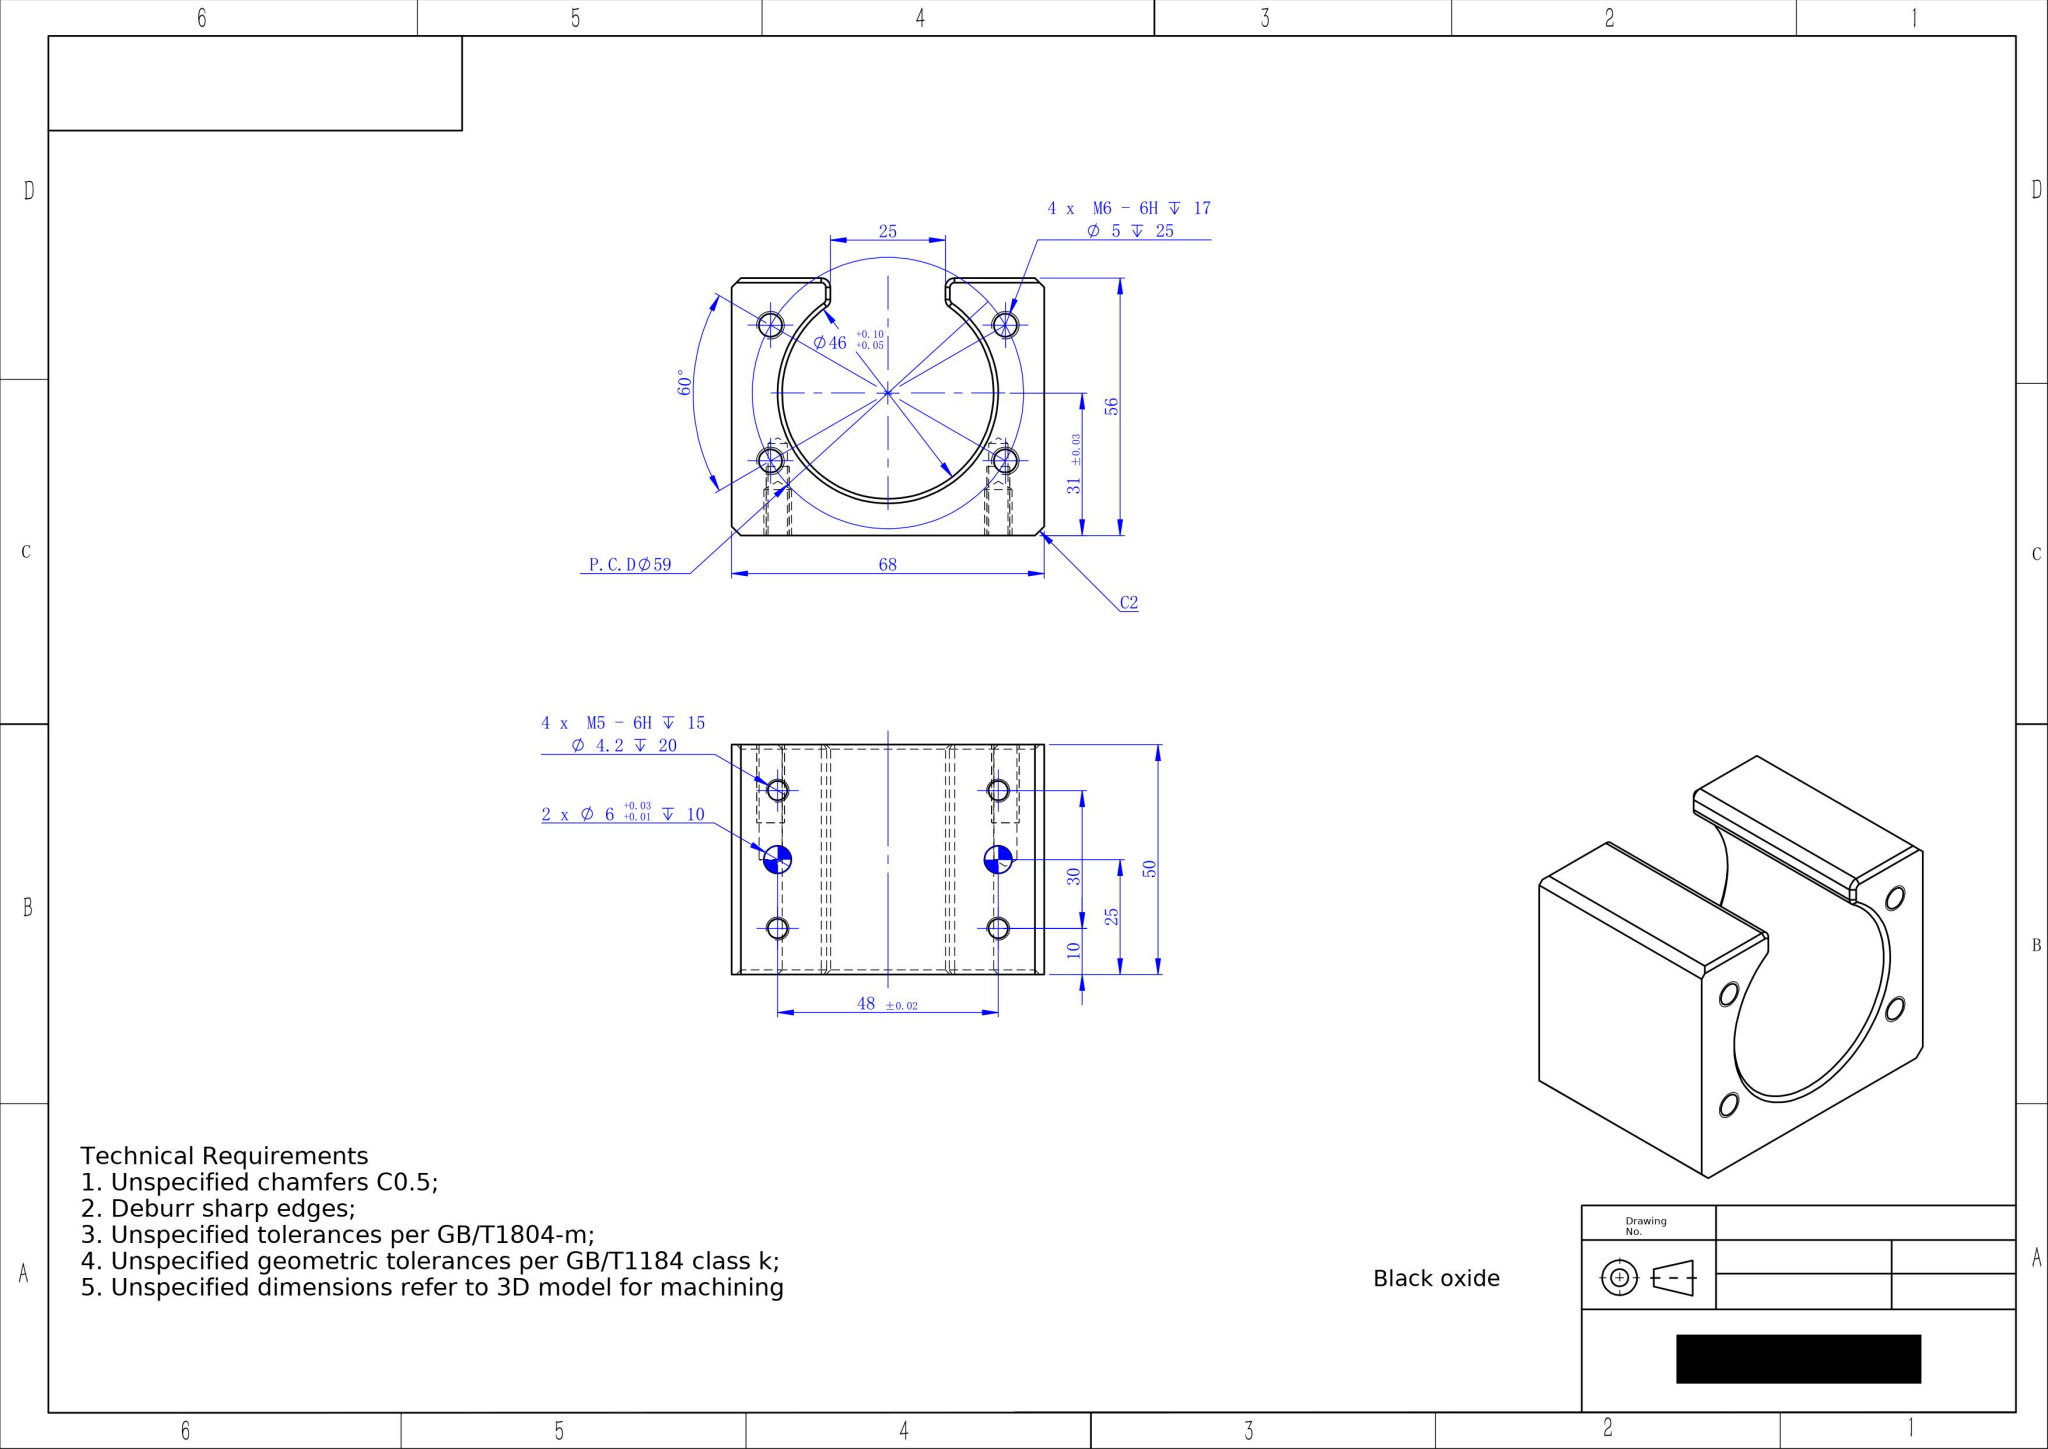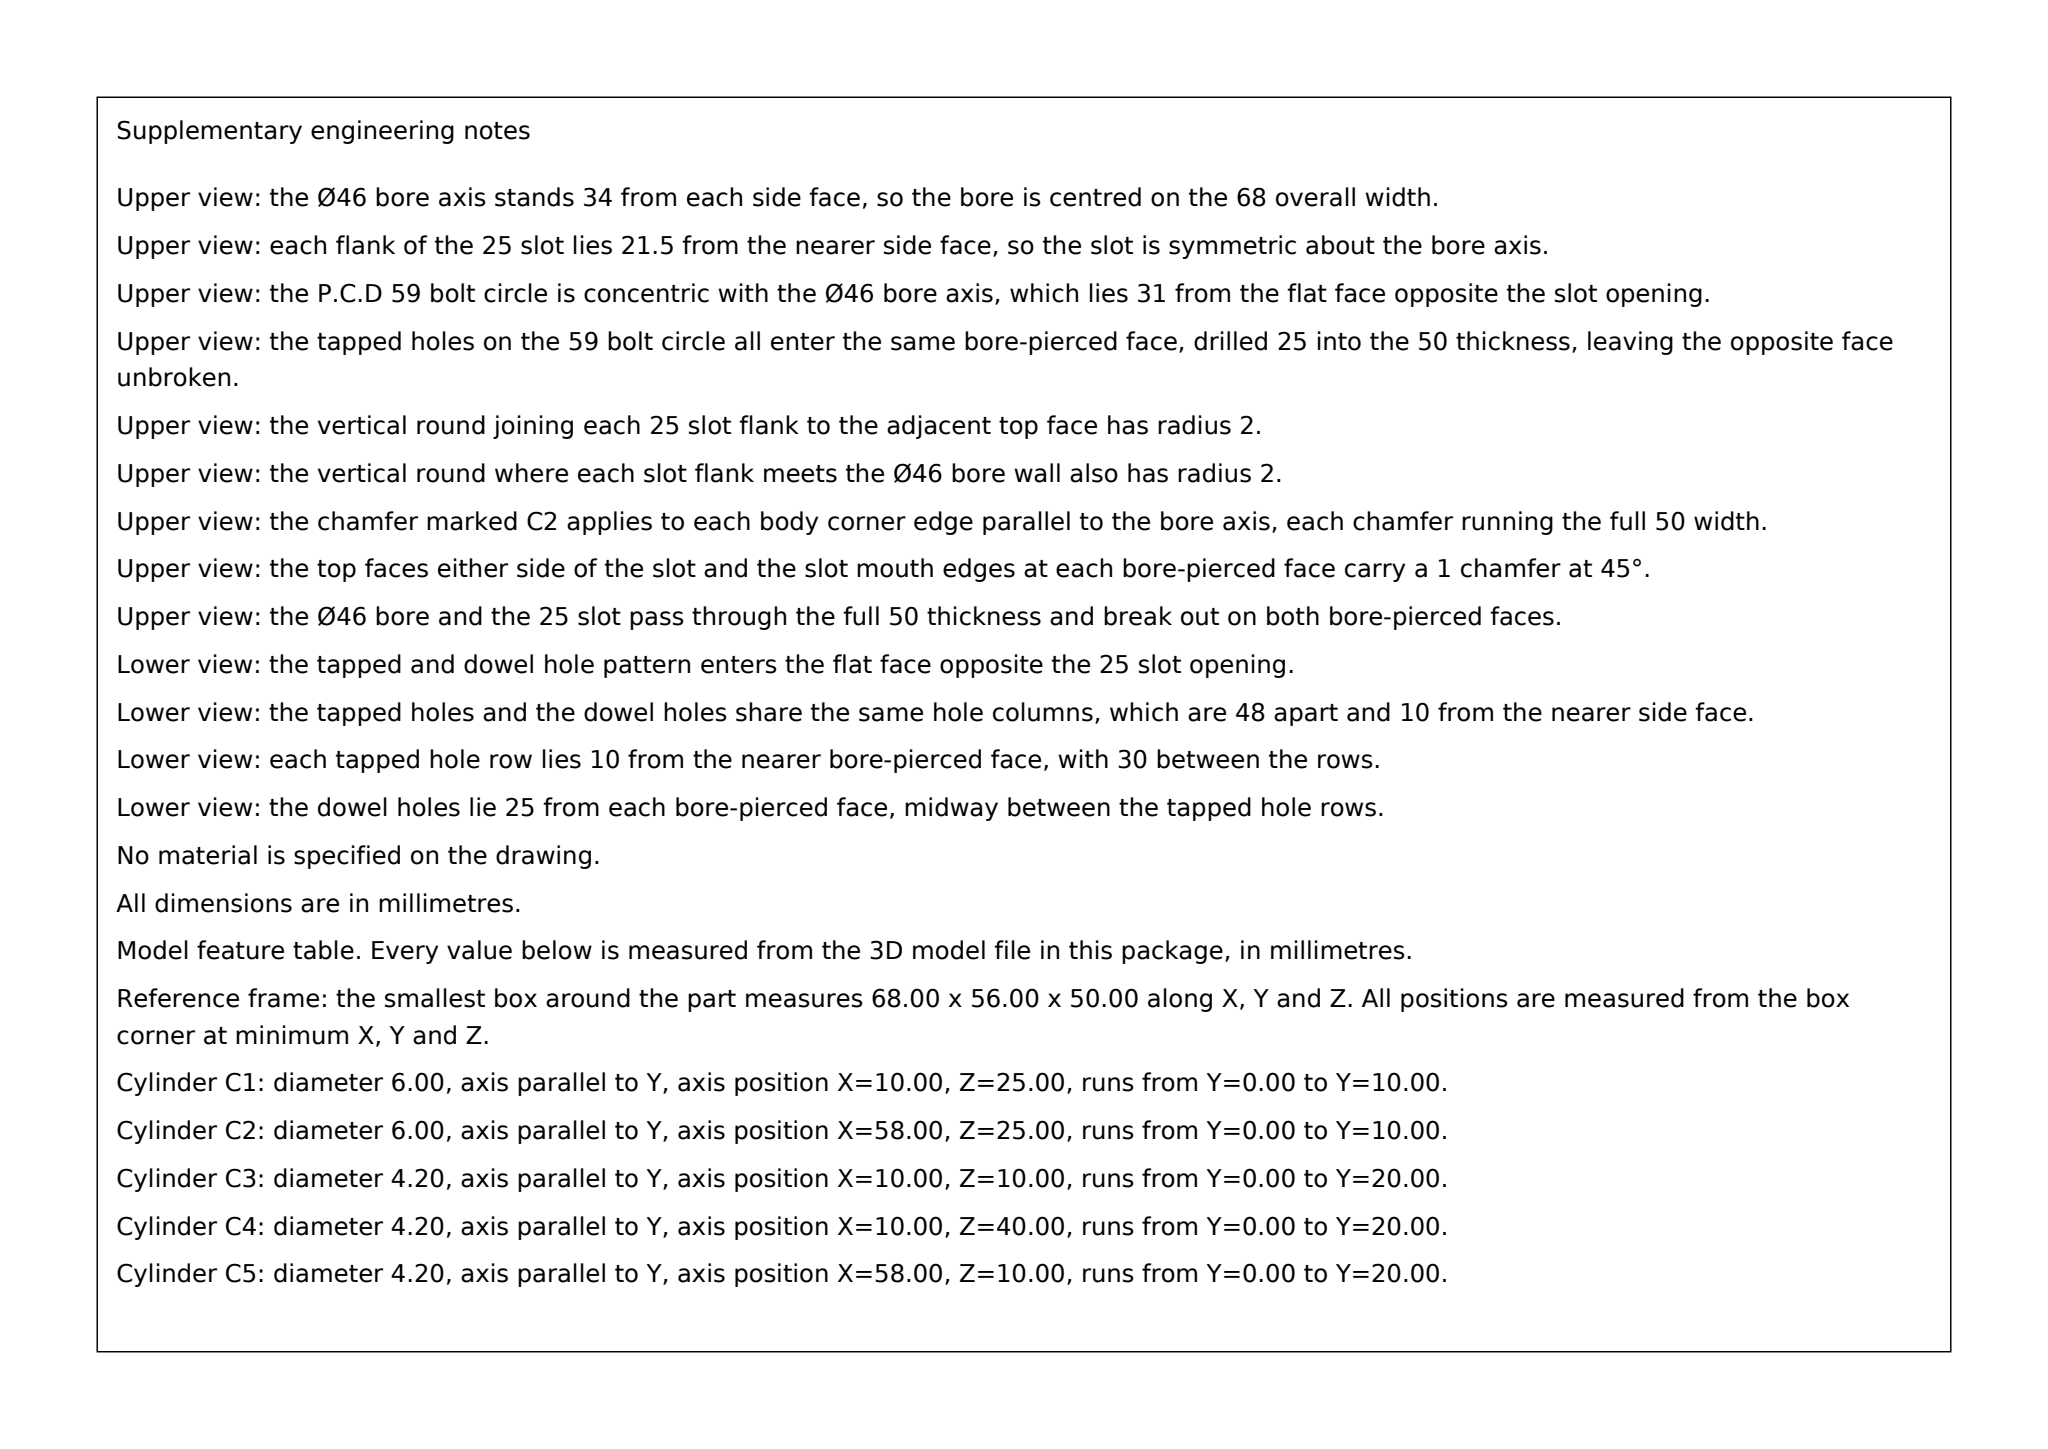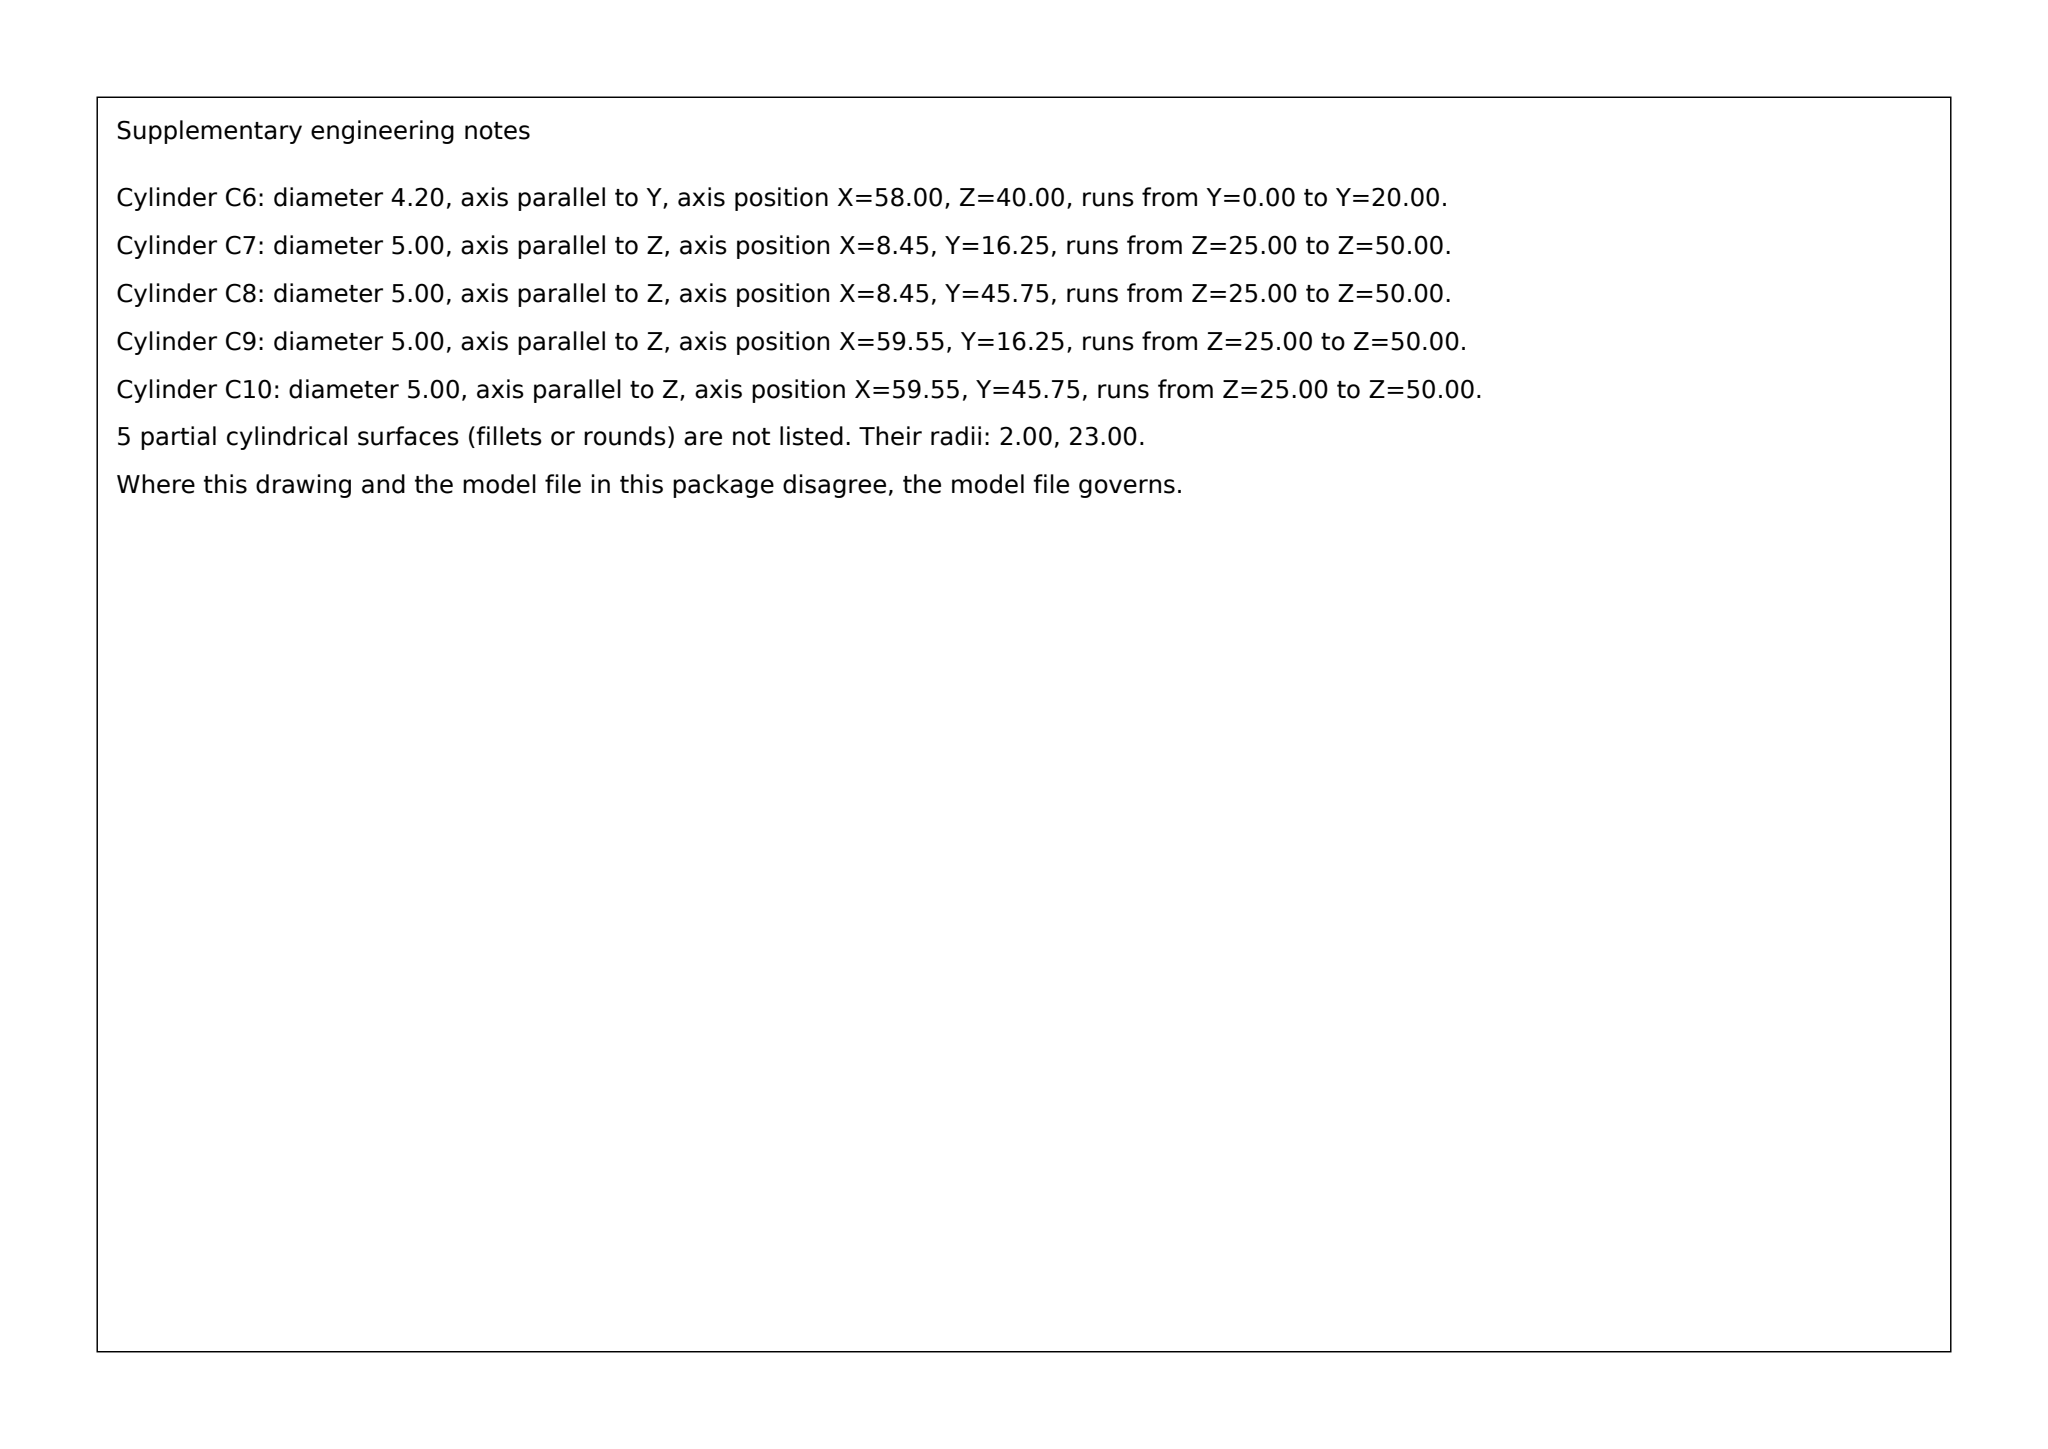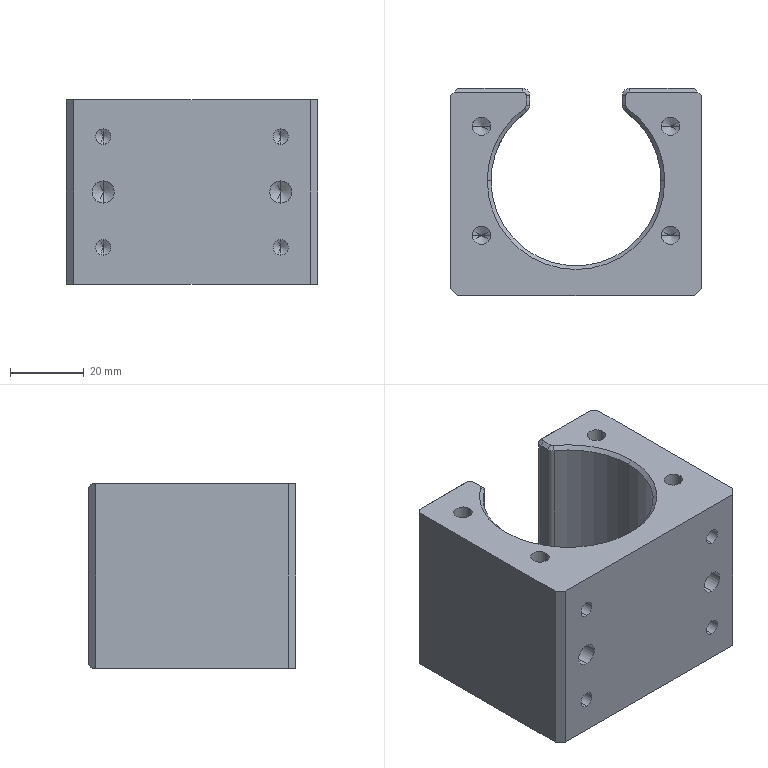Part | SolidWorks | mm | 1 solid | 84 faces | box 68 x 56 x 50 mm | volume 99002 mm3 | cone 34 | cylinder 29 | plane 21 | commonest cylinder face diameters 4.2 x10 5 x8 6 x4 4 x4 46 x3
Drawing notes:
Ø46 BORE: C1 x 45° BOTH ENDS (BORE CYL 48 LG IN 50 THK) | from the solid: Ø46 z-cyl len 48 in 50 thk bbox; cones 90° ref dia 48 & 46 at each end = 1 mm radial
M6-6H DP 17, Ø5 DP 25: 8X TOTAL, 4X EA FROM FRONT & REAR FACE | from the solid: Ø5 z-cyls len 25 at (8.45,16.25),(8.45,45.75),(59.55,16.25),(59.55,45.75) count 2 each = 8 holes in 50 thk part
M5-6H DP 15, Ø4.2 DP 20: 8X TOTAL, 4X EA FROM TOP & BOT FACE | from the solid: Ø4.2 y-cyls len 20 at x=10 & 58, z=10 & 40, count 2 each = 8 holes in 56 high part
Ø6 +0.03/+0.01 DP 10: 4X TOTAL, 2X EA FROM TOP & BOT FACE | from the solid: Ø6 y-cyls len 10 at (x=10,z=25) and (x=58,z=25), count 2 each = 4 holes
4X C2 CHAMFER AT BLOCK CORNERS, FRONT VIEW | from the solid: Front-view profile (68 x 56 block, planes x=0/68, y=0/56) shows 2 mm corner breaks at all four outer corners; no fillet radii present.